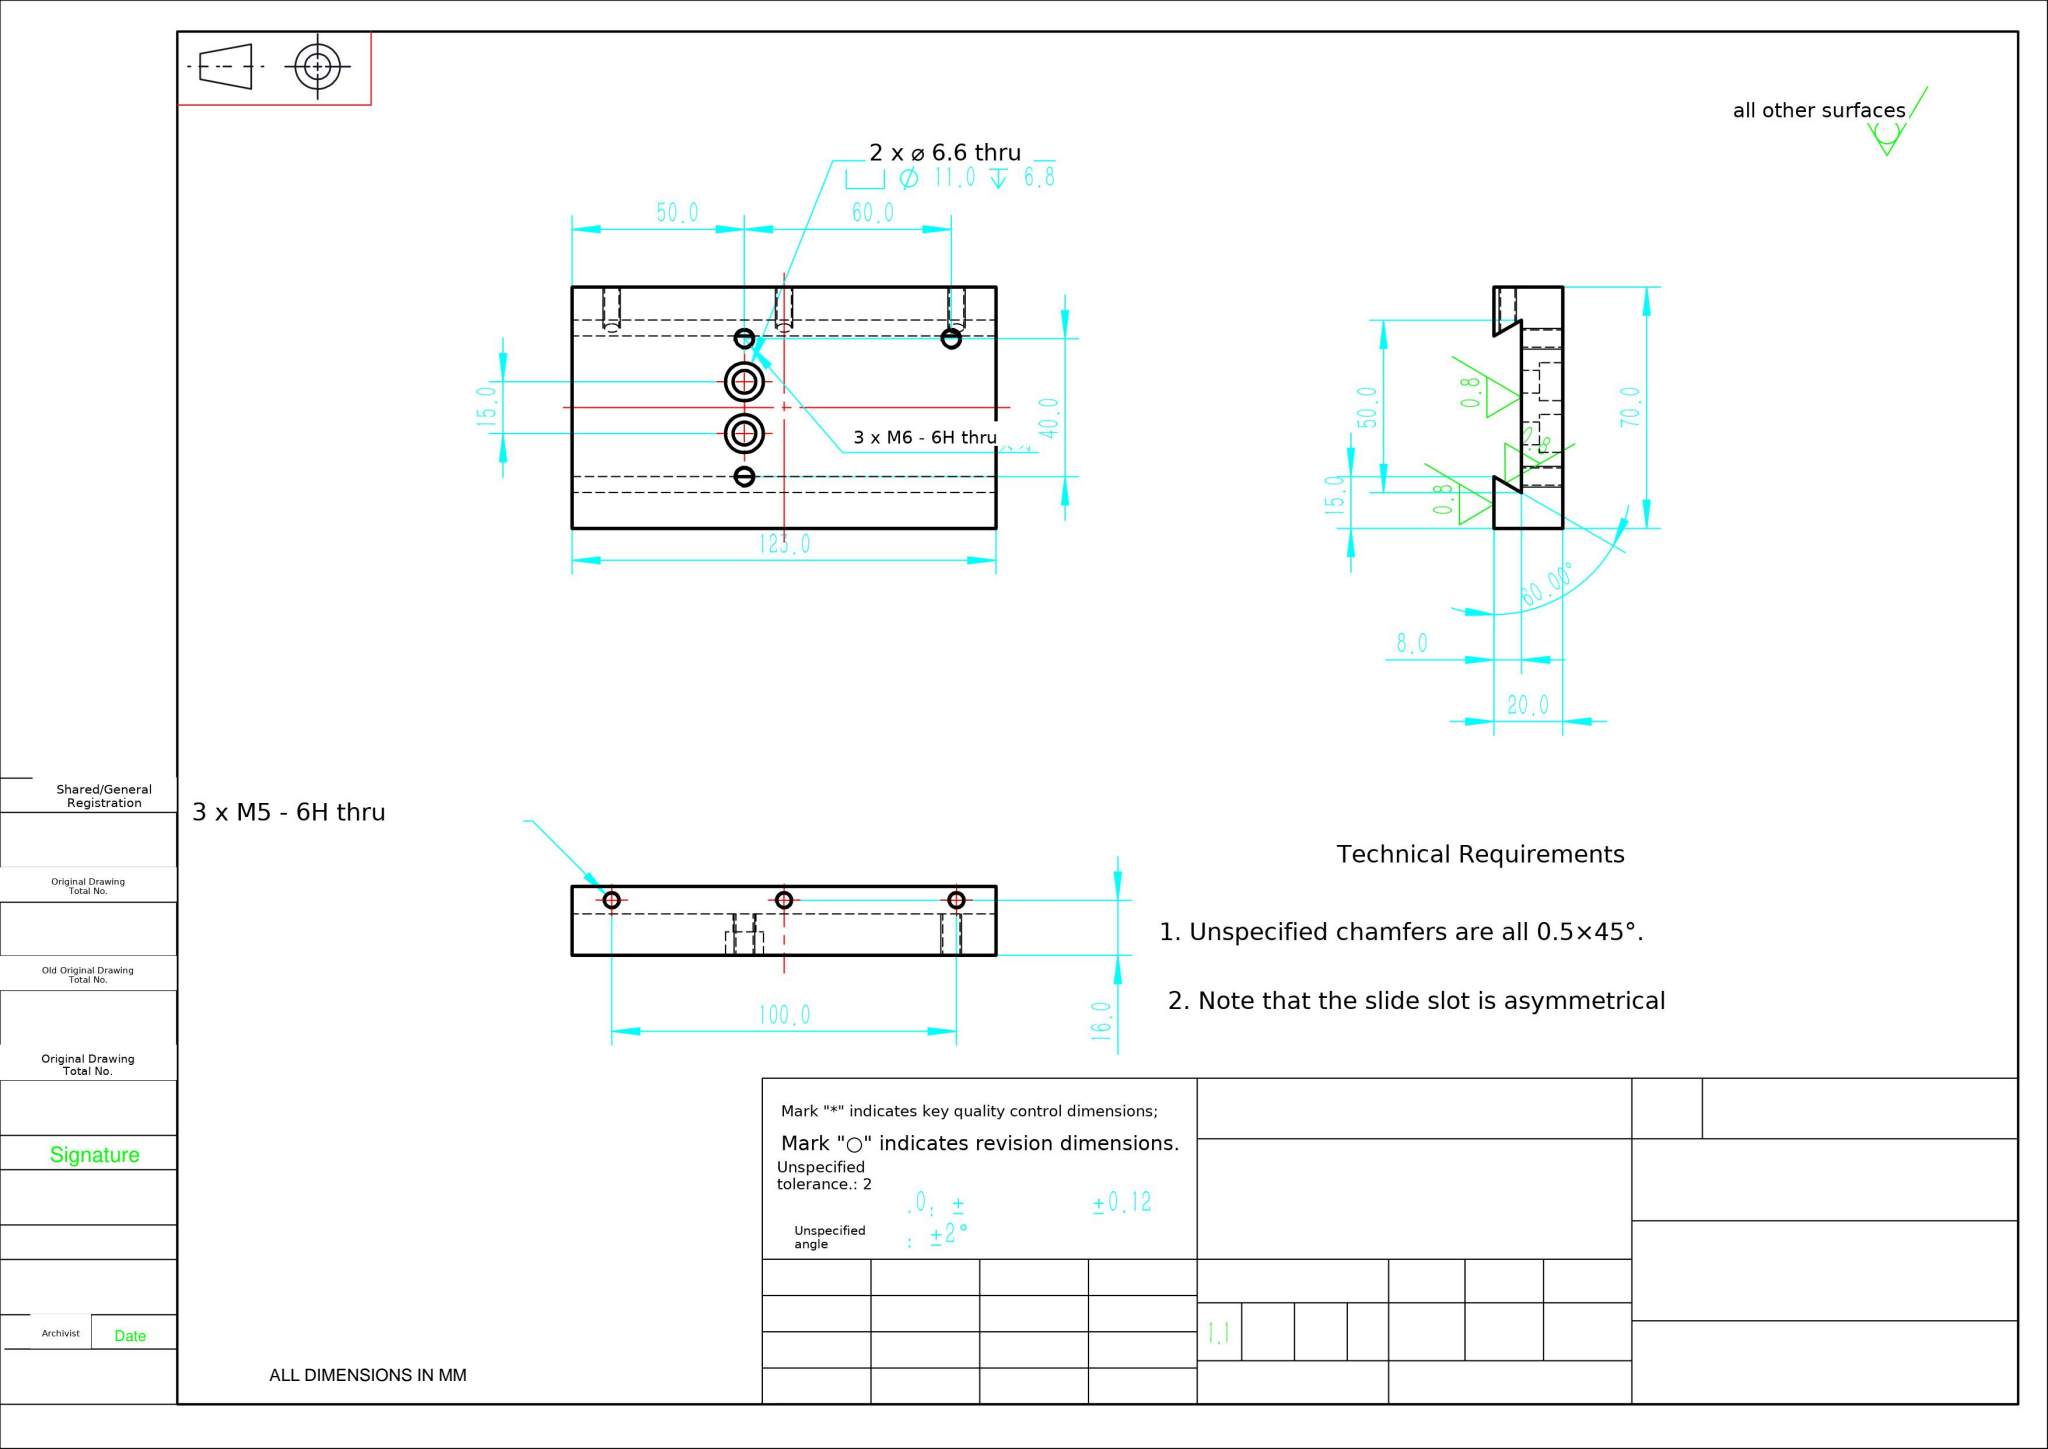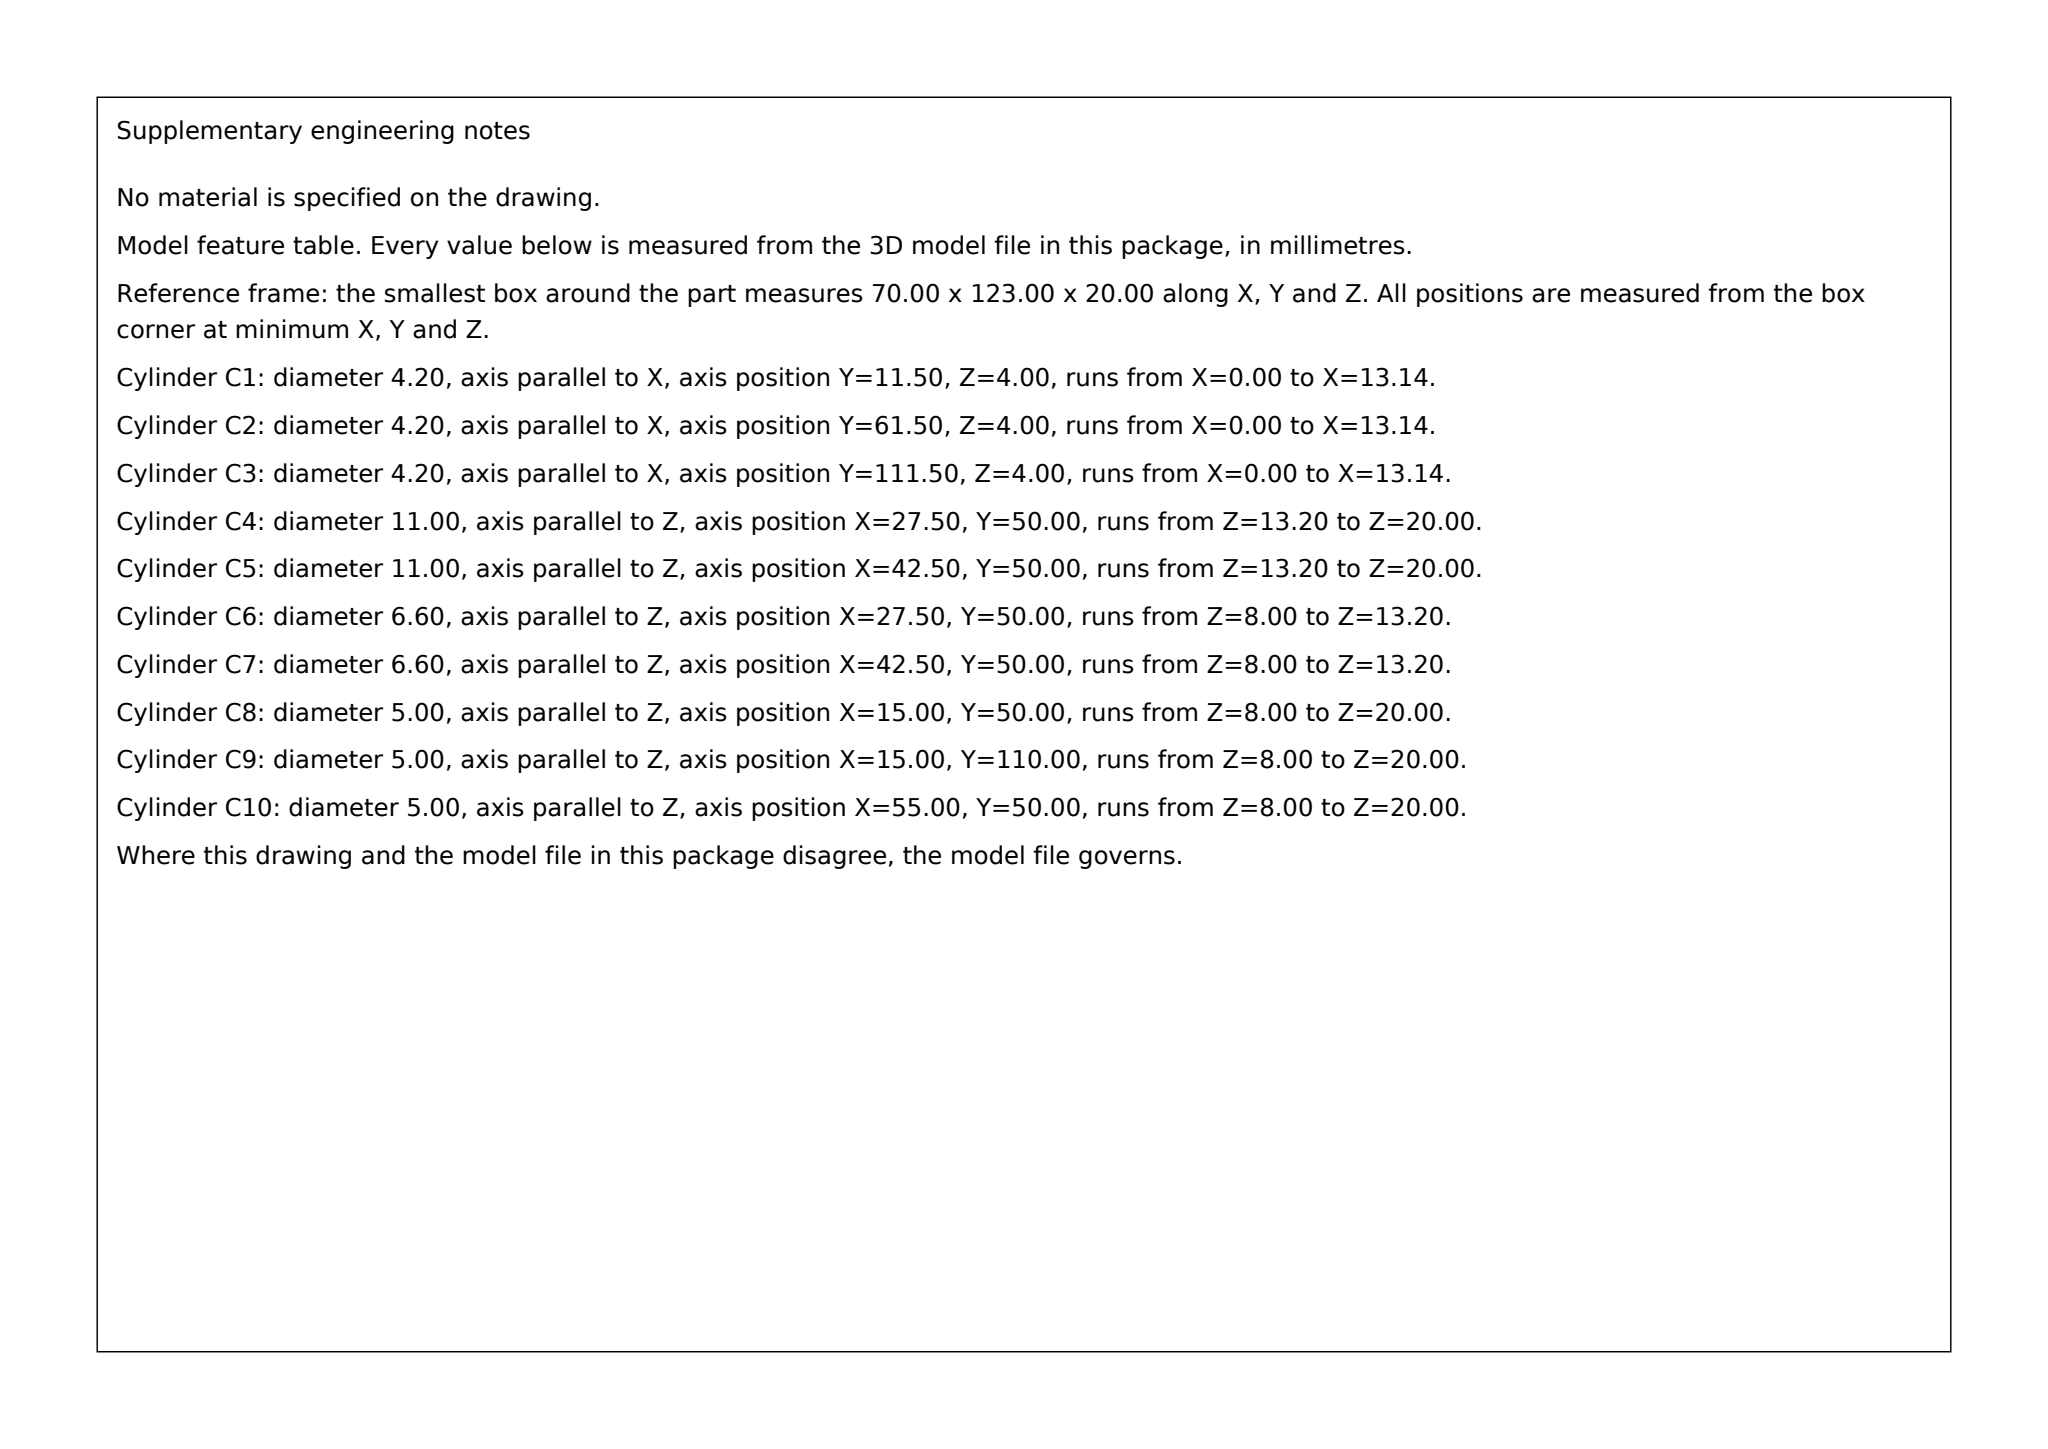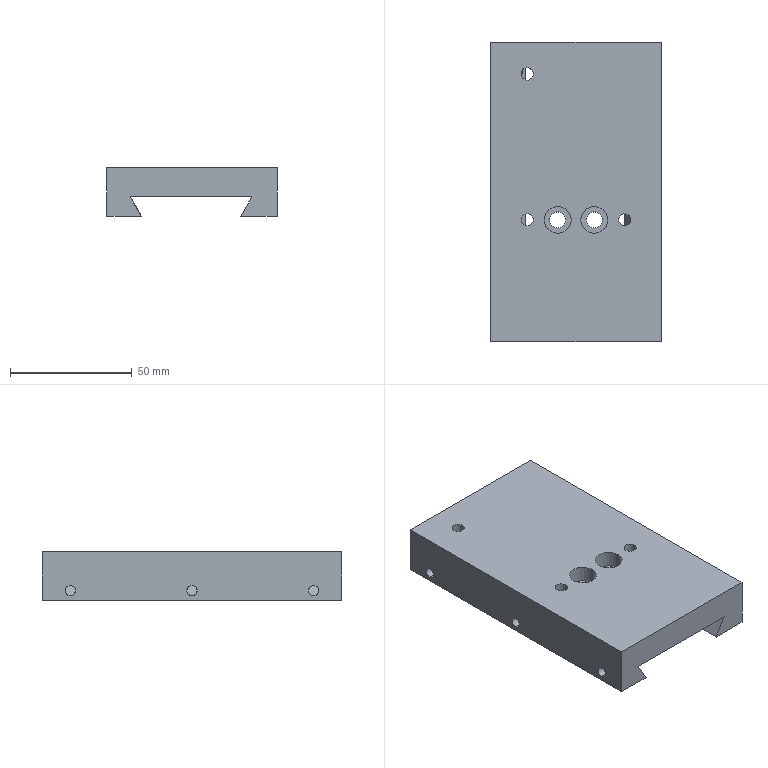Part | SolidWorks | mm | 1 solid | 32 faces | box 70 x 123 x 20 mm | volume 124694 mm3 | cylinder 20 | plane 12 | commonest cylinder face diameters 5 x6 4.2 x6 11 x4 6.6 x4
build123d program:
from build123d import *

# Parameters (mm, degrees)
BOSS_EXTRUDE1_DEPTH                               = 123
M5_TAPPED_HOLE1_REACH                             = 145.892
M5_TAPPED_HOLE1_BORE_R                            = 2.1
HOLE_SIZE_ACCORDING_TO_TYPE_1_OF_HEXA_D           = 6.6
HOLE_SIZE_ACCORDING_TO_TYPE_1_OF_HEXA_CBORE_D     = 11
HOLE_SIZE_ACCORDING_TO_TYPE_1_OF_HEXA_CBORE_DEPTH = 6.8
M6_TAPPED_HOLE2_D                                 = 5
M6_TAPPED_HOLE2_DEPTH                             = 12


with BuildPart() as part:
    # Sketch2 → Boss-Extrude1 (new body)
    with BuildSketch(Plane(origin=(0, 0, 0), x_dir=(1, 0, 0), z_dir=(0, 1, 0))):
        Polygon((63.867, -6), (78.104, -6), (73.486, -14), (123.486, -14), (118.867, -6), (133.867, -6), (133.867, -26), (63.867, -26), align=None)
    extrude(amount=BOSS_EXTRUDE1_DEPTH)

    # M5 Tapped Hole1 bore → M5 Tapped Hole1 (cut, up to next)
    with BuildSketch(Plane.ZY.offset(-63.867), mode=Mode.PRIVATE) as m5_tapped_hole1_sk1:
        with Locations((10, 11.5)):
            Circle(M5_TAPPED_HOLE1_BORE_R)
    m5_tapped_hole1_tool1 = extrude(m5_tapped_hole1_sk1.sketch, amount=-M5_TAPPED_HOLE1_REACH, mode=Mode.PRIVATE) & part.part
    # M5 Tapped Hole1 bore → M5 Tapped Hole1 (cut, up to next)
    with BuildSketch(Plane.ZY.offset(-63.867), mode=Mode.PRIVATE) as m5_tapped_hole1_sk2:
        with Locations((10, 61.5)):
            Circle(M5_TAPPED_HOLE1_BORE_R)
    m5_tapped_hole1_tool2 = extrude(m5_tapped_hole1_sk2.sketch, amount=-M5_TAPPED_HOLE1_REACH, mode=Mode.PRIVATE) & part.part
    # M5 Tapped Hole1 bore → M5 Tapped Hole1 (cut, up to next)
    with BuildSketch(Plane.ZY.offset(-63.867), mode=Mode.PRIVATE) as m5_tapped_hole1_sk3:
        with Locations((10, 111.5)):
            Circle(M5_TAPPED_HOLE1_BORE_R)
    m5_tapped_hole1_tool3 = extrude(m5_tapped_hole1_sk3.sketch, amount=-M5_TAPPED_HOLE1_REACH, mode=Mode.PRIVATE) & part.part
    add(m5_tapped_hole1_tool1.solids().sort_by_distance((63.867, 11.5, 10))[0], mode=Mode.SUBTRACT)
    add(m5_tapped_hole1_tool2.solids().sort_by_distance((63.867, 61.5, 10))[0], mode=Mode.SUBTRACT)
    add(m5_tapped_hole1_tool3.solids().sort_by_distance((63.867, 111.5, 10))[0], mode=Mode.SUBTRACT)

    # Hole Size _ according to_ Type 1 of Hexa (through all)
    with Locations(Plane.XY.offset(26)):
        with Locations((91.367, 50), (106.367, 50)):
            CounterBoreHole(HOLE_SIZE_ACCORDING_TO_TYPE_1_OF_HEXA_D / 2, HOLE_SIZE_ACCORDING_TO_TYPE_1_OF_HEXA_CBORE_D / 2, HOLE_SIZE_ACCORDING_TO_TYPE_1_OF_HEXA_CBORE_DEPTH)

    # M6 Tapped Hole2
    with Locations(Plane.XY.offset(26)):
        with Locations((78.867, 50), (78.867, 110), (118.867, 50)):
            Hole(M6_TAPPED_HOLE2_D / 2, depth=M6_TAPPED_HOLE2_DEPTH)


solid = part.part